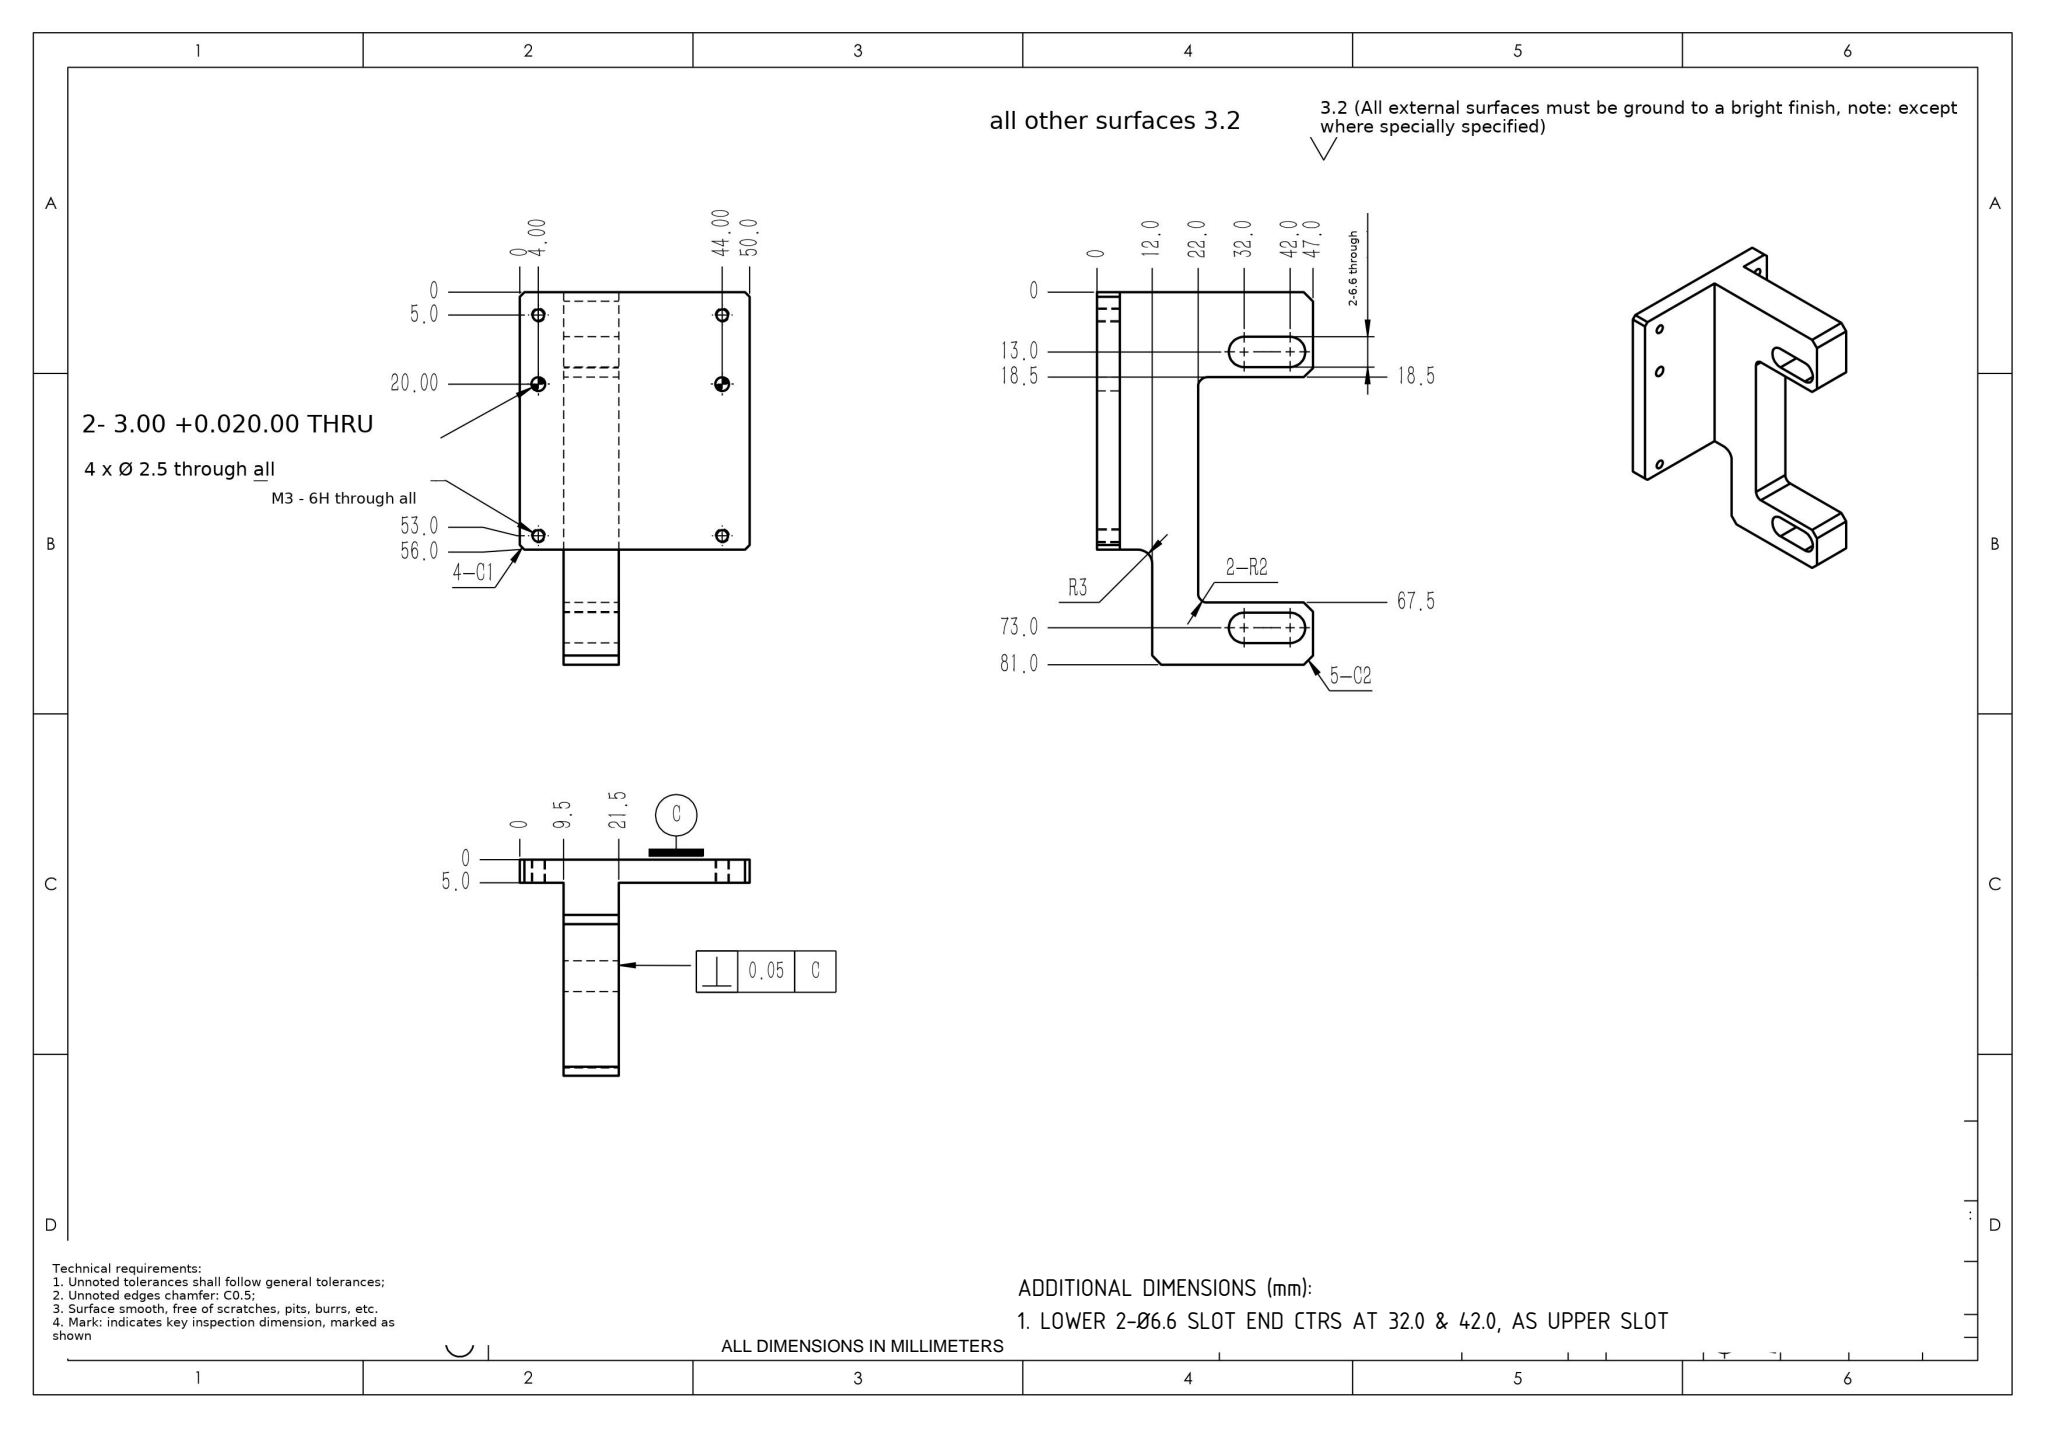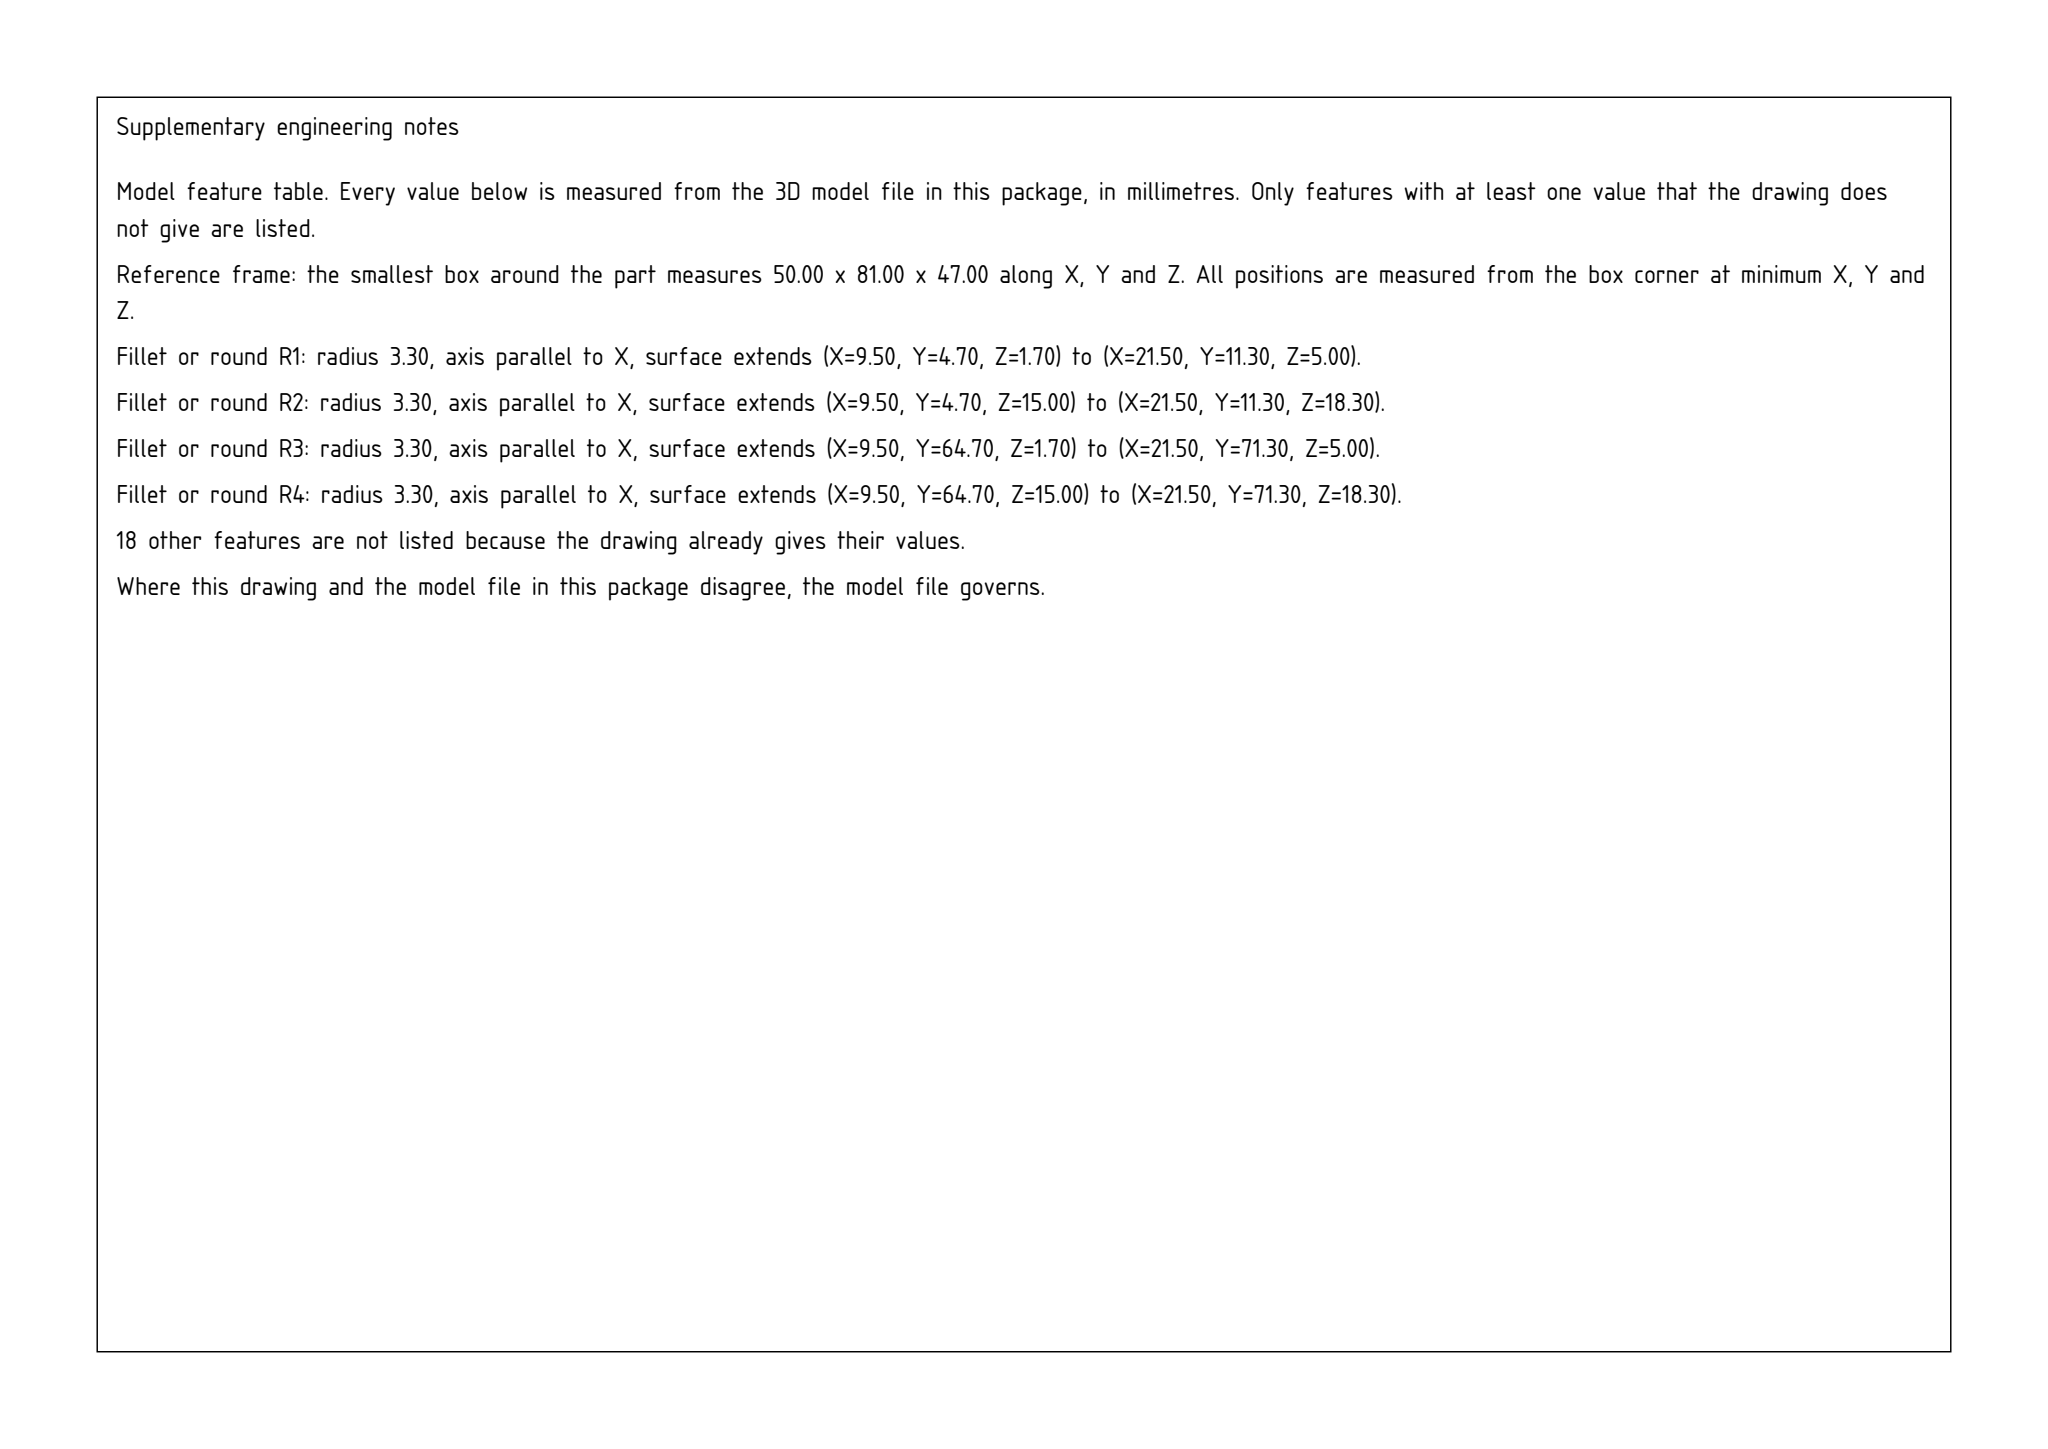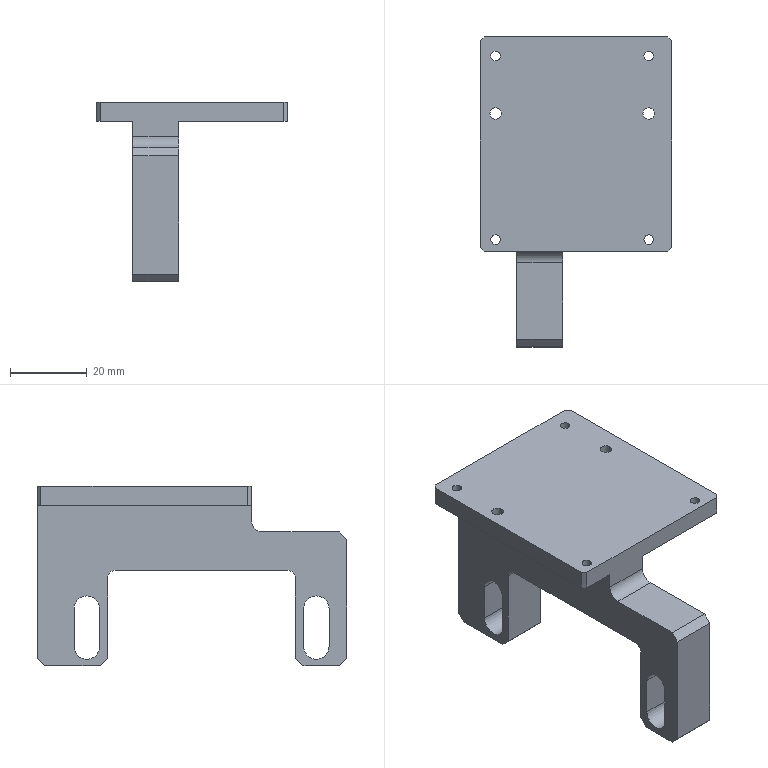Part | SolidWorks | mm | 1 solid | 50 faces | box 50 x 81 x 47 mm | volume 35364 mm3 | plane 29 | cylinder 21 | commonest cylinder face diameters 2.5 x8 6.6 x6 3 x4 4 x2 6 x1